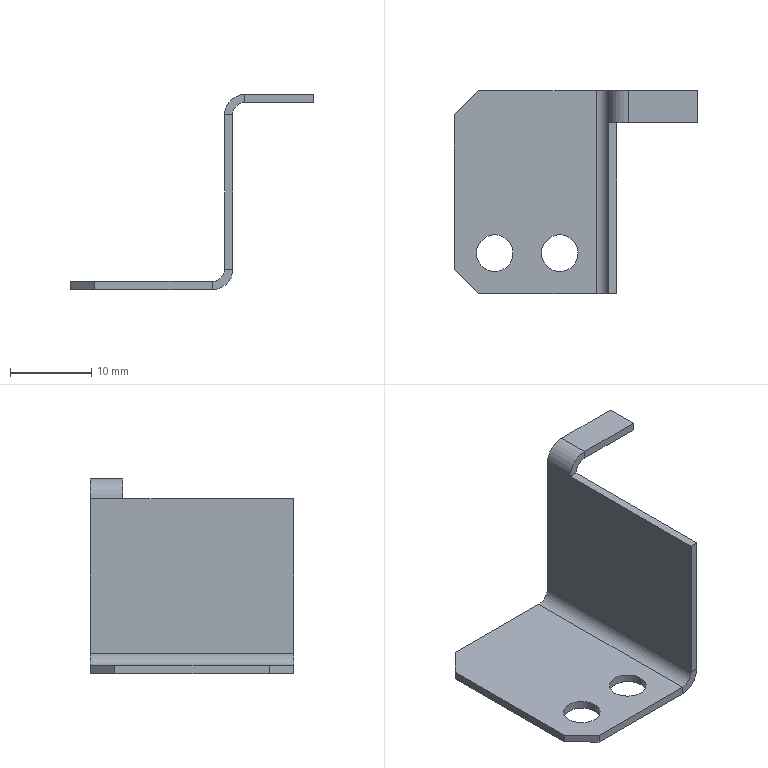Component | SolidWorks | F12529-S5108-2 | 1 solid | 29 faces | box 30 x 25 x 24 mm | volume 997 mm3 | plane 21 | cylinder 8 | commonest cylinder face diameters 4.5 x4 5 x2 3 x2
STEP:
#1=CARTESIAN_POINT('',(-1.467,7.795,1.201));
#2=VERTEX_POINT('',#1);
#3=CARTESIAN_POINT('',(-1.644,7.795,1.201));
#4=VERTEX_POINT('',#3);
#5=CARTESIAN_POINT('',(-1.555,7.795,1.201));
#6=DIRECTION('',(0.,0.,-1.));
#7=DIRECTION('',(-1.,0.,-0.));
#8=AXIS2_PLACEMENT_3D('',#5,#6,#7);
#9=CIRCLE('',#8,0.08858);
#10=EDGE_CURVE('',#2,#4,#9,.T.);
#11=ORIENTED_EDGE('',*,*,#10,.T.);
#12=CARTESIAN_POINT('',(-1.644,7.795,1.24));
#13=VERTEX_POINT('',#12);
#14=CARTESIAN_POINT('',(-1.644,7.795,0.8465));
#15=DIRECTION('',(-0.,0.,1.));
#16=VECTOR('',#15,39.37);
#17=LINE('',#14,#16);
#18=EDGE_CURVE('',#4,#13,#17,.T.);
#19=ORIENTED_EDGE('',*,*,#18,.T.);
#20=CARTESIAN_POINT('',(-1.467,7.795,1.24));
#21=VERTEX_POINT('',#20);
#22=CARTESIAN_POINT('',(-1.555,7.795,1.24));
#23=DIRECTION('',(-0.,0.,1.));
#24=DIRECTION('',(1.,0.,0.));
#25=AXIS2_PLACEMENT_3D('',#22,#23,#24);
#26=CIRCLE('',#25,0.08858);
#27=EDGE_CURVE('',#13,#21,#26,.T.);
#28=ORIENTED_EDGE('',*,*,#27,.T.);
#29=CARTESIAN_POINT('',(-1.467,7.795,0.8465));
#30=DIRECTION('',(-0.,0.,1.));
#31=VECTOR('',#30,39.37);
#32=LINE('',#29,#31);
#33=EDGE_CURVE('',#2,#21,#32,.T.);
#34=ORIENTED_EDGE('',*,*,#33,.F.);
#35=EDGE_LOOP('',(#11,#19,#28,#34));
#36=FACE_OUTER_BOUND('',#35,.T.);
#37=CARTESIAN_POINT('',(-1.555,7.795,0.8465));
#38=DIRECTION('',(-0.,0.,1.));
#39=DIRECTION('',(1.,0.,0.));
#40=AXIS2_PLACEMENT_3D('',#37,#38,#39);
#41=CYLINDRICAL_SURFACE('',#40,0.08858);
#42=ADVANCED_FACE('',(#36),#41,.F.);
#43=CARTESIAN_POINT('',(-1.781,7.795,1.201));
#44=VERTEX_POINT('',#43);
#45=CARTESIAN_POINT('',(-1.959,7.795,1.201));
#46=VERTEX_POINT('',#45);
#47=CARTESIAN_POINT('',(-1.87,7.795,1.201));
#48=DIRECTION('',(0.,0.,-1.));
#49=DIRECTION('',(-1.,0.,-0.));
#50=AXIS2_PLACEMENT_3D('',#47,#48,#49);
#51=CIRCLE('',#50,0.08858);
#52=EDGE_CURVE('',#44,#46,#51,.T.);
#53=ORIENTED_EDGE('',*,*,#52,.T.);
#54=CARTESIAN_POINT('',(-1.959,7.795,1.24));
#55=VERTEX_POINT('',#54);
#56=CARTESIAN_POINT('',(-1.959,7.795,0.8465));
#57=DIRECTION('',(-0.,0.,1.));
#58=VECTOR('',#57,39.37);
#59=LINE('',#56,#58);
#60=EDGE_CURVE('',#46,#55,#59,.T.);
#61=ORIENTED_EDGE('',*,*,#60,.T.);
#62=CARTESIAN_POINT('',(-1.781,7.795,1.24));
#63=VERTEX_POINT('',#62);
#64=CARTESIAN_POINT('',(-1.87,7.795,1.24));
#65=DIRECTION('',(-0.,0.,1.));
#66=DIRECTION('',(1.,0.,0.));
#67=AXIS2_PLACEMENT_3D('',#64,#65,#66);
#68=CIRCLE('',#67,0.08858);
#69=EDGE_CURVE('',#55,#63,#68,.T.);
#70=ORIENTED_EDGE('',*,*,#69,.T.);
#71=CARTESIAN_POINT('',(-1.781,7.795,0.8465));
#72=DIRECTION('',(-0.,0.,1.));
#73=VECTOR('',#72,39.37);
#74=LINE('',#71,#73);
#75=EDGE_CURVE('',#44,#63,#74,.T.);
#76=ORIENTED_EDGE('',*,*,#75,.F.);
#77=EDGE_LOOP('',(#53,#61,#70,#76));
#78=FACE_OUTER_BOUND('',#77,.T.);
#79=CARTESIAN_POINT('',(-1.87,7.795,0.8465));
#80=DIRECTION('',(-0.,0.,1.));
#81=DIRECTION('',(1.,0.,0.));
#82=AXIS2_PLACEMENT_3D('',#79,#80,#81);
#83=CYLINDRICAL_SURFACE('',#82,0.08858);
#84=ADVANCED_FACE('',(#78),#83,.F.);
#85=CARTESIAN_POINT('',(-1.28,8.583,1.299));
#86=VERTEX_POINT('',#85);
#87=CARTESIAN_POINT('',(-1.319,8.583,1.299));
#88=VERTEX_POINT('',#87);
#89=CARTESIAN_POINT('',(-1.28,8.583,1.299));
#90=DIRECTION('',(-1.,0.,-0.));
#91=VECTOR('',#90,39.37);
#92=LINE('',#89,#91);
#93=EDGE_CURVE('',#86,#88,#92,.T.);
#94=ORIENTED_EDGE('',*,*,#93,.F.);
#95=CARTESIAN_POINT('',(-1.378,8.583,1.201));
#96=VERTEX_POINT('',#95);
#97=CARTESIAN_POINT('',(-1.378,8.583,1.299));
#98=DIRECTION('',(0.,-1.,0.));
#99=DIRECTION('',(-1.,0.,0.));
#100=AXIS2_PLACEMENT_3D('',#97,#98,#99);
#101=CIRCLE('',#100,0.09843);
#102=EDGE_CURVE('',#96,#86,#101,.T.);
#103=ORIENTED_EDGE('',*,*,#102,.F.);
#104=CARTESIAN_POINT('',(-1.378,8.583,1.24));
#105=VERTEX_POINT('',#104);
#106=CARTESIAN_POINT('',(-1.378,8.583,1.24));
#107=DIRECTION('',(0.,0.,-1.));
#108=VECTOR('',#107,39.37);
#109=LINE('',#106,#108);
#110=EDGE_CURVE('',#105,#96,#109,.T.);
#111=ORIENTED_EDGE('',*,*,#110,.F.);
#112=CARTESIAN_POINT('',(-1.378,8.583,1.299));
#113=DIRECTION('',(0.,-1.,0.));
#114=DIRECTION('',(0.,0.,1.));
#115=AXIS2_PLACEMENT_3D('',#112,#113,#114);
#116=CIRCLE('',#115,0.05906);
#117=EDGE_CURVE('',#105,#88,#116,.T.);
#118=ORIENTED_EDGE('',*,*,#117,.T.);
#119=EDGE_LOOP('',(#94,#103,#111,#118));
#120=FACE_OUTER_BOUND('',#119,.T.);
#121=CARTESIAN_POINT('',(-1.28,8.583,1.299));
#122=DIRECTION('',(0.,1.,0.));
#123=DIRECTION('',(-1.,0.,-0.));
#124=AXIS2_PLACEMENT_3D('',#121,#122,#123);
#125=PLANE('',#124);
#126=ADVANCED_FACE('',(#120),#125,.T.);
#127=CARTESIAN_POINT('',(-1.28,8.583,2.047));
#128=VERTEX_POINT('',#127);
#129=CARTESIAN_POINT('',(-1.28,8.583,1.201));
#130=DIRECTION('',(-0.,0.,1.));
#131=VECTOR('',#130,39.37);
#132=LINE('',#129,#131);
#133=EDGE_CURVE('',#86,#128,#132,.T.);
#134=ORIENTED_EDGE('',*,*,#133,.F.);
#135=ORIENTED_EDGE('',*,*,#93,.T.);
#136=CARTESIAN_POINT('',(-1.319,8.583,2.047));
#137=VERTEX_POINT('',#136);
#138=CARTESIAN_POINT('',(-1.319,8.583,1.201));
#139=DIRECTION('',(-0.,0.,1.));
#140=VECTOR('',#139,39.37);
#141=LINE('',#138,#140);
#142=EDGE_CURVE('',#88,#137,#141,.T.);
#143=ORIENTED_EDGE('',*,*,#142,.T.);
#144=CARTESIAN_POINT('',(-1.319,8.583,2.047));
#145=DIRECTION('',(1.,0.,0.));
#146=VECTOR('',#145,39.37);
#147=LINE('',#144,#146);
#148=EDGE_CURVE('',#137,#128,#147,.T.);
#149=ORIENTED_EDGE('',*,*,#148,.T.);
#150=EDGE_LOOP('',(#134,#135,#143,#149));
#151=FACE_OUTER_BOUND('',#150,.T.);
#152=CARTESIAN_POINT('',(-1.378,8.583,1.24));
#153=DIRECTION('',(0.,1.,0.));
#154=DIRECTION('',(-1.,0.,-0.));
#155=AXIS2_PLACEMENT_3D('',#152,#153,#154);
#156=PLANE('',#155);
#157=ADVANCED_FACE('',(#151),#156,.T.);
#158=CARTESIAN_POINT('',(-1.378,7.598,1.201));
#159=VERTEX_POINT('',#158);
#160=CARTESIAN_POINT('',(-1.378,7.598,1.24));
#161=VERTEX_POINT('',#160);
#162=CARTESIAN_POINT('',(-1.378,7.598,1.201));
#163=DIRECTION('',(-0.,0.,1.));
#164=VECTOR('',#163,39.37);
#165=LINE('',#162,#164);
#166=EDGE_CURVE('',#159,#161,#165,.T.);
#167=ORIENTED_EDGE('',*,*,#166,.F.);
#168=CARTESIAN_POINT('',(-1.28,7.598,1.299));
#169=VERTEX_POINT('',#168);
#170=CARTESIAN_POINT('',(-1.378,7.598,1.299));
#171=DIRECTION('',(0.,-1.,0.));
#172=DIRECTION('',(-1.,0.,0.));
#173=AXIS2_PLACEMENT_3D('',#170,#171,#172);
#174=CIRCLE('',#173,0.09843);
#175=EDGE_CURVE('',#159,#169,#174,.T.);
#176=ORIENTED_EDGE('',*,*,#175,.T.);
#177=CARTESIAN_POINT('',(-1.319,7.598,1.299));
#178=VERTEX_POINT('',#177);
#179=CARTESIAN_POINT('',(-1.319,7.598,1.299));
#180=DIRECTION('',(1.,0.,0.));
#181=VECTOR('',#180,39.37);
#182=LINE('',#179,#181);
#183=EDGE_CURVE('',#178,#169,#182,.T.);
#184=ORIENTED_EDGE('',*,*,#183,.F.);
#185=CARTESIAN_POINT('',(-1.378,7.598,1.299));
#186=DIRECTION('',(0.,-1.,0.));
#187=DIRECTION('',(0.,0.,1.));
#188=AXIS2_PLACEMENT_3D('',#185,#186,#187);
#189=CIRCLE('',#188,0.05906);
#190=EDGE_CURVE('',#161,#178,#189,.T.);
#191=ORIENTED_EDGE('',*,*,#190,.F.);
#192=EDGE_LOOP('',(#167,#176,#184,#191));
#193=FACE_OUTER_BOUND('',#192,.T.);
#194=CARTESIAN_POINT('',(-1.378,7.598,1.201));
#195=DIRECTION('',(0.,-1.,0.));
#196=DIRECTION('',(1.,0.,0.));
#197=AXIS2_PLACEMENT_3D('',#194,#195,#196);
#198=PLANE('',#197);
#199=ADVANCED_FACE('',(#193),#198,.T.);
#200=CARTESIAN_POINT('',(-1.949,7.598,1.24));
#201=VERTEX_POINT('',#200);
#202=CARTESIAN_POINT('',(-2.067,7.598,1.24));
#203=DIRECTION('',(1.,0.,0.));
#204=VECTOR('',#203,39.37);
#205=LINE('',#202,#204);
#206=EDGE_CURVE('',#201,#161,#205,.T.);
#207=ORIENTED_EDGE('',*,*,#206,.F.);
#208=CARTESIAN_POINT('',(-1.949,7.598,1.201));
#209=VERTEX_POINT('',#208);
#210=CARTESIAN_POINT('',(-1.949,7.598,1.299));
#211=DIRECTION('',(0.,0.,-1.));
#212=VECTOR('',#211,39.37);
#213=LINE('',#210,#212);
#214=EDGE_CURVE('',#201,#209,#213,.T.);
#215=ORIENTED_EDGE('',*,*,#214,.T.);
#216=CARTESIAN_POINT('',(-2.067,7.598,1.201));
#217=DIRECTION('',(1.,0.,0.));
#218=VECTOR('',#217,39.37);
#219=LINE('',#216,#218);
#220=EDGE_CURVE('',#209,#159,#219,.T.);
#221=ORIENTED_EDGE('',*,*,#220,.T.);
#222=ORIENTED_EDGE('',*,*,#166,.T.);
#223=EDGE_LOOP('',(#207,#215,#221,#222));
#224=FACE_OUTER_BOUND('',#223,.T.);
#225=CARTESIAN_POINT('',(-1.319,7.598,1.299));
#226=DIRECTION('',(0.,-1.,0.));
#227=DIRECTION('',(1.,0.,0.));
#228=AXIS2_PLACEMENT_3D('',#225,#226,#227);
#229=PLANE('',#228);
#230=ADVANCED_FACE('',(#224),#229,.T.);
#231=CARTESIAN_POINT('',(-1.28,7.598,2.047));
#232=VERTEX_POINT('',#231);
#233=CARTESIAN_POINT('',(-1.28,7.598,1.201));
#234=DIRECTION('',(-0.,0.,1.));
#235=VECTOR('',#234,39.37);
#236=LINE('',#233,#235);
#237=EDGE_CURVE('',#169,#232,#236,.T.);
#238=ORIENTED_EDGE('',*,*,#237,.T.);
#239=CARTESIAN_POINT('',(-1.319,7.598,2.047));
#240=VERTEX_POINT('',#239);
#241=CARTESIAN_POINT('',(-1.28,7.598,2.047));
#242=DIRECTION('',(-1.,0.,-0.));
#243=VECTOR('',#242,39.37);
#244=LINE('',#241,#243);
#245=EDGE_CURVE('',#232,#240,#244,.T.);
#246=ORIENTED_EDGE('',*,*,#245,.T.);
#247=CARTESIAN_POINT('',(-1.319,7.598,1.201));
#248=DIRECTION('',(-0.,0.,1.));
#249=VECTOR('',#248,39.37);
#250=LINE('',#247,#249);
#251=EDGE_CURVE('',#178,#240,#250,.T.);
#252=ORIENTED_EDGE('',*,*,#251,.F.);
#253=ORIENTED_EDGE('',*,*,#183,.T.);
#254=EDGE_LOOP('',(#238,#246,#252,#253));
#255=FACE_OUTER_BOUND('',#254,.T.);
#256=CARTESIAN_POINT('',(-1.22,7.598,2.146));
#257=DIRECTION('',(0.,-1.,0.));
#258=DIRECTION('',(1.,0.,0.));
#259=AXIS2_PLACEMENT_3D('',#256,#257,#258);
#260=PLANE('',#259);
#261=ADVANCED_FACE('',(#255),#260,.T.);
#262=ORIENTED_EDGE('',*,*,#237,.F.);
#263=CARTESIAN_POINT('',(-1.28,8.583,1.299));
#264=DIRECTION('',(0.,-1.,0.));
#265=VECTOR('',#264,39.37);
#266=LINE('',#263,#265);
#267=EDGE_CURVE('',#86,#169,#266,.T.);
#268=ORIENTED_EDGE('',*,*,#267,.F.);
#269=ORIENTED_EDGE('',*,*,#133,.T.);
#270=CARTESIAN_POINT('',(-1.28,8.425,2.047));
#271=VERTEX_POINT('',#270);
#272=CARTESIAN_POINT('',(-1.28,8.583,2.047));
#273=DIRECTION('',(0.,-1.,0.));
#274=VECTOR('',#273,39.37);
#275=LINE('',#272,#274);
#276=EDGE_CURVE('',#128,#271,#275,.T.);
#277=ORIENTED_EDGE('',*,*,#276,.T.);
#278=CARTESIAN_POINT('',(-1.28,7.598,2.047));
#279=DIRECTION('',(0.,-1.,0.));
#280=VECTOR('',#279,39.37);
#281=LINE('',#278,#280);
#282=EDGE_CURVE('',#271,#232,#281,.T.);
#283=ORIENTED_EDGE('',*,*,#282,.T.);
#284=EDGE_LOOP('',(#262,#268,#269,#277,#283));
#285=FACE_OUTER_BOUND('',#284,.T.);
#286=CARTESIAN_POINT('',(-1.28,8.583,1.201));
#287=DIRECTION('',(1.,0.,0.));
#288=DIRECTION('',(0.,0.,-1.));
#289=AXIS2_PLACEMENT_3D('',#286,#287,#288);
#290=PLANE('',#289);
#291=ADVANCED_FACE('',(#285),#290,.T.);
#292=ORIENTED_EDGE('',*,*,#175,.F.);
#293=CARTESIAN_POINT('',(-1.378,8.583,1.201));
#294=DIRECTION('',(0.,-1.,0.));
#295=VECTOR('',#294,39.37);
#296=LINE('',#293,#295);
#297=EDGE_CURVE('',#96,#159,#296,.T.);
#298=ORIENTED_EDGE('',*,*,#297,.F.);
#299=ORIENTED_EDGE('',*,*,#102,.T.);
#300=ORIENTED_EDGE('',*,*,#267,.T.);
#301=EDGE_LOOP('',(#292,#298,#299,#300));
#302=FACE_OUTER_BOUND('',#301,.T.);
#303=CARTESIAN_POINT('',(-1.378,8.583,1.299));
#304=DIRECTION('',(0.,-1.,0.));
#305=DIRECTION('',(1.,0.,0.));
#306=AXIS2_PLACEMENT_3D('',#303,#304,#305);
#307=CYLINDRICAL_SURFACE('',#306,0.09843);
#308=ADVANCED_FACE('',(#302),#307,.T.);
#309=ORIENTED_EDGE('',*,*,#10,.F.);
#310=CARTESIAN_POINT('',(-1.555,7.795,1.201));
#311=DIRECTION('',(0.,0.,-1.));
#312=DIRECTION('',(-1.,0.,-0.));
#313=AXIS2_PLACEMENT_3D('',#310,#311,#312);
#314=CIRCLE('',#313,0.08858);
#315=EDGE_CURVE('',#4,#2,#314,.T.);
#316=ORIENTED_EDGE('',*,*,#315,.F.);
#317=EDGE_LOOP('',(#309,#316));
#318=FACE_BOUND('',#317,.T.);
#319=ORIENTED_EDGE('',*,*,#52,.F.);
#320=CARTESIAN_POINT('',(-1.87,7.795,1.201));
#321=DIRECTION('',(0.,0.,-1.));
#322=DIRECTION('',(-1.,0.,-0.));
#323=AXIS2_PLACEMENT_3D('',#320,#321,#322);
#324=CIRCLE('',#323,0.08858);
#325=EDGE_CURVE('',#46,#44,#324,.T.);
#326=ORIENTED_EDGE('',*,*,#325,.F.);
#327=EDGE_LOOP('',(#319,#326));
#328=FACE_BOUND('',#327,.T.);
#329=ORIENTED_EDGE('',*,*,#220,.F.);
#330=CARTESIAN_POINT('',(-2.067,7.717,1.201));
#331=VERTEX_POINT('',#330);
#332=CARTESIAN_POINT('',(-2.5,8.15,1.201));
#333=DIRECTION('',(-0.7071,0.7071,-0.));
#334=VECTOR('',#333,39.37);
#335=LINE('',#332,#334);
#336=EDGE_CURVE('',#209,#331,#335,.T.);
#337=ORIENTED_EDGE('',*,*,#336,.T.);
#338=CARTESIAN_POINT('',(-2.067,8.465,1.201));
#339=VERTEX_POINT('',#338);
#340=CARTESIAN_POINT('',(-2.067,8.583,1.201));
#341=DIRECTION('',(0.,-1.,0.));
#342=VECTOR('',#341,39.37);
#343=LINE('',#340,#342);
#344=EDGE_CURVE('',#339,#331,#343,.T.);
#345=ORIENTED_EDGE('',*,*,#344,.F.);
#346=CARTESIAN_POINT('',(-1.949,8.583,1.201));
#347=VERTEX_POINT('',#346);
#348=CARTESIAN_POINT('',(-2.008,8.524,1.201));
#349=DIRECTION('',(0.7071,0.7071,0.));
#350=VECTOR('',#349,39.37);
#351=LINE('',#348,#350);
#352=EDGE_CURVE('',#339,#347,#351,.T.);
#353=ORIENTED_EDGE('',*,*,#352,.T.);
#354=CARTESIAN_POINT('',(-2.067,8.583,1.201));
#355=DIRECTION('',(1.,0.,0.));
#356=VECTOR('',#355,39.37);
#357=LINE('',#354,#356);
#358=EDGE_CURVE('',#347,#96,#357,.T.);
#359=ORIENTED_EDGE('',*,*,#358,.T.);
#360=ORIENTED_EDGE('',*,*,#297,.T.);
#361=EDGE_LOOP('',(#329,#337,#345,#353,#359,#360));
#362=FACE_OUTER_BOUND('',#361,.T.);
#363=CARTESIAN_POINT('',(-2.067,8.583,1.201));
#364=DIRECTION('',(0.,0.,-1.));
#365=DIRECTION('',(-1.,0.,-0.));
#366=AXIS2_PLACEMENT_3D('',#363,#364,#365);
#367=PLANE('',#366);
#368=ADVANCED_FACE('',(#318,#328,#362),#367,.T.);
#369=ORIENTED_EDGE('',*,*,#344,.T.);
#370=CARTESIAN_POINT('',(-2.067,7.717,1.24));
#371=VERTEX_POINT('',#370);
#372=CARTESIAN_POINT('',(-2.067,7.717,1.24));
#373=DIRECTION('',(-0.,0.,1.));
#374=VECTOR('',#373,39.37);
#375=LINE('',#372,#374);
#376=EDGE_CURVE('',#331,#371,#375,.T.);
#377=ORIENTED_EDGE('',*,*,#376,.T.);
#378=CARTESIAN_POINT('',(-2.067,8.465,1.24));
#379=VERTEX_POINT('',#378);
#380=CARTESIAN_POINT('',(-2.067,8.583,1.24));
#381=DIRECTION('',(0.,-1.,0.));
#382=VECTOR('',#381,39.37);
#383=LINE('',#380,#382);
#384=EDGE_CURVE('',#379,#371,#383,.T.);
#385=ORIENTED_EDGE('',*,*,#384,.F.);
#386=CARTESIAN_POINT('',(-2.067,8.465,1.201));
#387=DIRECTION('',(0.,0.,-1.));
#388=VECTOR('',#387,39.37);
#389=LINE('',#386,#388);
#390=EDGE_CURVE('',#379,#339,#389,.T.);
#391=ORIENTED_EDGE('',*,*,#390,.T.);
#392=EDGE_LOOP('',(#369,#377,#385,#391));
#393=FACE_OUTER_BOUND('',#392,.T.);
#394=CARTESIAN_POINT('',(-2.067,8.583,1.24));
#395=DIRECTION('',(-1.,0.,-0.));
#396=DIRECTION('',(-0.,0.,1.));
#397=AXIS2_PLACEMENT_3D('',#394,#395,#396);
#398=PLANE('',#397);
#399=ADVANCED_FACE('',(#393),#398,.T.);
#400=CARTESIAN_POINT('',(-1.555,7.795,1.24));
#401=DIRECTION('',(-0.,0.,1.));
#402=DIRECTION('',(1.,0.,0.));
#403=AXIS2_PLACEMENT_3D('',#400,#401,#402);
#404=CIRCLE('',#403,0.08858);
#405=EDGE_CURVE('',#21,#13,#404,.T.);
#406=ORIENTED_EDGE('',*,*,#405,.F.);
#407=ORIENTED_EDGE('',*,*,#27,.F.);
#408=EDGE_LOOP('',(#406,#407));
#409=FACE_BOUND('',#408,.T.);
#410=CARTESIAN_POINT('',(-1.87,7.795,1.24));
#411=DIRECTION('',(-0.,0.,1.));
#412=DIRECTION('',(1.,0.,0.));
#413=AXIS2_PLACEMENT_3D('',#410,#411,#412);
#414=CIRCLE('',#413,0.08858);
#415=EDGE_CURVE('',#63,#55,#414,.T.);
#416=ORIENTED_EDGE('',*,*,#415,.F.);
#417=ORIENTED_EDGE('',*,*,#69,.F.);
#418=EDGE_LOOP('',(#416,#417));
#419=FACE_BOUND('',#418,.T.);
#420=ORIENTED_EDGE('',*,*,#384,.T.);
#421=CARTESIAN_POINT('',(-1.949,7.598,1.24));
#422=DIRECTION('',(0.7071,-0.7071,0.));
#423=VECTOR('',#422,39.37);
#424=LINE('',#421,#423);
#425=EDGE_CURVE('',#371,#201,#424,.T.);
#426=ORIENTED_EDGE('',*,*,#425,.T.);
#427=ORIENTED_EDGE('',*,*,#206,.T.);
#428=CARTESIAN_POINT('',(-1.378,8.583,1.24));
#429=DIRECTION('',(0.,-1.,0.));
#430=VECTOR('',#429,39.37);
#431=LINE('',#428,#430);
#432=EDGE_CURVE('',#105,#161,#431,.T.);
#433=ORIENTED_EDGE('',*,*,#432,.F.);
#434=CARTESIAN_POINT('',(-1.949,8.583,1.24));
#435=VERTEX_POINT('',#434);
#436=CARTESIAN_POINT('',(-2.067,8.583,1.24));
#437=DIRECTION('',(1.,0.,0.));
#438=VECTOR('',#437,39.37);
#439=LINE('',#436,#438);
#440=EDGE_CURVE('',#435,#105,#439,.T.);
#441=ORIENTED_EDGE('',*,*,#440,.F.);
#442=CARTESIAN_POINT('',(-2.067,8.465,1.24));
#443=DIRECTION('',(-0.7071,-0.7071,-0.));
#444=VECTOR('',#443,39.37);
#445=LINE('',#442,#444);
#446=EDGE_CURVE('',#435,#379,#445,.T.);
#447=ORIENTED_EDGE('',*,*,#446,.T.);
#448=EDGE_LOOP('',(#420,#426,#427,#433,#441,#447));
#449=FACE_OUTER_BOUND('',#448,.T.);
#450=CARTESIAN_POINT('',(-2.067,8.583,1.24));
#451=DIRECTION('',(0.,0.,-1.));
#452=DIRECTION('',(-1.,0.,-0.));
#453=AXIS2_PLACEMENT_3D('',#450,#451,#452);
#454=PLANE('',#453);
#455=ADVANCED_FACE('',(#409,#419,#449),#454,.F.);
#456=ORIENTED_EDGE('',*,*,#190,.T.);
#457=CARTESIAN_POINT('',(-1.319,8.583,1.299));
#458=DIRECTION('',(0.,-1.,0.));
#459=VECTOR('',#458,39.37);
#460=LINE('',#457,#459);
#461=EDGE_CURVE('',#88,#178,#460,.T.);
#462=ORIENTED_EDGE('',*,*,#461,.F.);
#463=ORIENTED_EDGE('',*,*,#117,.F.);
#464=ORIENTED_EDGE('',*,*,#432,.T.);
#465=EDGE_LOOP('',(#456,#462,#463,#464));
#466=FACE_OUTER_BOUND('',#465,.T.);
#467=CARTESIAN_POINT('',(-1.378,8.583,1.299));
#468=DIRECTION('',(0.,-1.,0.));
#469=DIRECTION('',(1.,0.,0.));
#470=AXIS2_PLACEMENT_3D('',#467,#468,#469);
#471=CYLINDRICAL_SURFACE('',#470,0.05906);
#472=ADVANCED_FACE('',(#466),#471,.F.);
#473=ORIENTED_EDGE('',*,*,#251,.T.);
#474=CARTESIAN_POINT('',(-1.319,8.425,2.047));
#475=VERTEX_POINT('',#474);
#476=CARTESIAN_POINT('',(-1.319,7.598,2.047));
#477=DIRECTION('',(0.,-1.,0.));
#478=VECTOR('',#477,39.37);
#479=LINE('',#476,#478);
#480=EDGE_CURVE('',#475,#240,#479,.T.);
#481=ORIENTED_EDGE('',*,*,#480,.F.);
#482=CARTESIAN_POINT('',(-1.319,8.583,2.047));
#483=DIRECTION('',(0.,-1.,0.));
#484=VECTOR('',#483,39.37);
#485=LINE('',#482,#484);
#486=EDGE_CURVE('',#137,#475,#485,.T.);
#487=ORIENTED_EDGE('',*,*,#486,.F.);
#488=ORIENTED_EDGE('',*,*,#142,.F.);
#489=ORIENTED_EDGE('',*,*,#461,.T.);
#490=EDGE_LOOP('',(#473,#481,#487,#488,#489));
#491=FACE_OUTER_BOUND('',#490,.T.);
#492=CARTESIAN_POINT('',(-1.319,8.583,1.201));
#493=DIRECTION('',(1.,0.,0.));
#494=DIRECTION('',(0.,0.,-1.));
#495=AXIS2_PLACEMENT_3D('',#492,#493,#494);
#496=PLANE('',#495);
#497=ADVANCED_FACE('',(#491),#496,.F.);
#498=ORIENTED_EDGE('',*,*,#358,.F.);
#499=CARTESIAN_POINT('',(-1.949,8.583,1.24));
#500=DIRECTION('',(-0.,0.,1.));
#501=VECTOR('',#500,39.37);
#502=LINE('',#499,#501);
#503=EDGE_CURVE('',#347,#435,#502,.T.);
#504=ORIENTED_EDGE('',*,*,#503,.T.);
#505=ORIENTED_EDGE('',*,*,#440,.T.);
#506=ORIENTED_EDGE('',*,*,#110,.T.);
#507=EDGE_LOOP('',(#498,#504,#505,#506));
#508=FACE_OUTER_BOUND('',#507,.T.);
#509=CARTESIAN_POINT('',(-1.22,8.583,2.047));
#510=DIRECTION('',(0.,-1.,0.));
#511=DIRECTION('',(0.,0.,-1.));
#512=AXIS2_PLACEMENT_3D('',#509,#510,#511);
#513=PLANE('',#512);
#514=ADVANCED_FACE('',(#508),#513,.F.);
#515=ORIENTED_EDGE('',*,*,#425,.F.);
#516=ORIENTED_EDGE('',*,*,#376,.F.);
#517=ORIENTED_EDGE('',*,*,#336,.F.);
#518=ORIENTED_EDGE('',*,*,#214,.F.);
#519=EDGE_LOOP('',(#515,#516,#517,#518));
#520=FACE_OUTER_BOUND('',#519,.T.);
#521=CARTESIAN_POINT('',(-1.949,7.598,1.299));
#522=DIRECTION('',(0.7071,0.7071,0.));
#523=DIRECTION('',(-0.7071,0.7071,-0.));
#524=AXIS2_PLACEMENT_3D('',#521,#522,#523);
#525=PLANE('',#524);
#526=ADVANCED_FACE('',(#520),#525,.F.);
#527=ORIENTED_EDGE('',*,*,#446,.F.);
#528=ORIENTED_EDGE('',*,*,#503,.F.);
#529=ORIENTED_EDGE('',*,*,#352,.F.);
#530=ORIENTED_EDGE('',*,*,#390,.F.);
#531=EDGE_LOOP('',(#527,#528,#529,#530));
#532=FACE_OUTER_BOUND('',#531,.T.);
#533=CARTESIAN_POINT('',(-2.067,8.465,1.24));
#534=DIRECTION('',(-0.7071,0.7071,-0.));
#535=DIRECTION('',(-0.7071,-0.7071,-0.));
#536=AXIS2_PLACEMENT_3D('',#533,#534,#535);
#537=PLANE('',#536);
#538=ADVANCED_FACE('',(#532),#537,.T.);
#539=ORIENTED_EDGE('',*,*,#480,.T.);
#540=ORIENTED_EDGE('',*,*,#245,.F.);
#541=ORIENTED_EDGE('',*,*,#282,.F.);
#542=CARTESIAN_POINT('',(-1.28,8.425,2.047));
#543=DIRECTION('',(-1.,0.,-0.));
#544=VECTOR('',#543,39.37);
#545=LINE('',#542,#544);
#546=EDGE_CURVE('',#271,#475,#545,.T.);
#547=ORIENTED_EDGE('',*,*,#546,.T.);
#548=EDGE_LOOP('',(#539,#540,#541,#547));
#549=FACE_OUTER_BOUND('',#548,.T.);
#550=CARTESIAN_POINT('',(-1.28,7.598,2.047));
#551=DIRECTION('',(0.,0.,-1.));
#552=DIRECTION('',(-1.,0.,-0.));
#553=AXIS2_PLACEMENT_3D('',#550,#551,#552);
#554=PLANE('',#553);
#555=ADVANCED_FACE('',(#549),#554,.F.);
#556=CARTESIAN_POINT('',(-1.22,8.425,2.106));
#557=VERTEX_POINT('',#556);
#558=CARTESIAN_POINT('',(-1.22,8.425,2.146));
#559=VERTEX_POINT('',#558);
#560=CARTESIAN_POINT('',(-1.22,8.425,2.106));
#561=DIRECTION('',(-0.,0.,1.));
#562=VECTOR('',#561,39.37);
#563=LINE('',#560,#562);
#564=EDGE_CURVE('',#557,#559,#563,.T.);
#565=ORIENTED_EDGE('',*,*,#564,.T.);
#566=CARTESIAN_POINT('',(-1.22,8.425,2.047));
#567=DIRECTION('',(0.,-1.,0.));
#568=DIRECTION('',(1.,0.,0.));
#569=AXIS2_PLACEMENT_3D('',#566,#567,#568);
#570=CIRCLE('',#569,0.09843);
#571=EDGE_CURVE('',#559,#475,#570,.T.);
#572=ORIENTED_EDGE('',*,*,#571,.T.);
#573=ORIENTED_EDGE('',*,*,#546,.F.);
#574=CARTESIAN_POINT('',(-1.22,8.425,2.047));
#575=DIRECTION('',(0.,-1.,0.));
#576=DIRECTION('',(1.,0.,0.));
#577=AXIS2_PLACEMENT_3D('',#574,#575,#576);
#578=CIRCLE('',#577,0.05906);
#579=EDGE_CURVE('',#557,#271,#578,.T.);
#580=ORIENTED_EDGE('',*,*,#579,.F.);
#581=EDGE_LOOP('',(#565,#572,#573,#580));
#582=FACE_OUTER_BOUND('',#581,.T.);
#583=CARTESIAN_POINT('',(-1.22,8.425,2.047));
#584=DIRECTION('',(0.,1.,0.));
#585=DIRECTION('',(-1.,0.,-0.));
#586=AXIS2_PLACEMENT_3D('',#583,#584,#585);
#587=PLANE('',#586);
#588=ADVANCED_FACE('',(#582),#587,.F.);
#589=ORIENTED_EDGE('',*,*,#148,.F.);
#590=CARTESIAN_POINT('',(-1.22,8.583,2.146));
#591=VERTEX_POINT('',#590);
#592=CARTESIAN_POINT('',(-1.22,8.583,2.047));
#593=DIRECTION('',(0.,1.,0.));
#594=DIRECTION('',(1.,0.,0.));
#595=AXIS2_PLACEMENT_3D('',#592,#593,#594);
#596=CIRCLE('',#595,0.09843);
#597=EDGE_CURVE('',#137,#591,#596,.T.);
#598=ORIENTED_EDGE('',*,*,#597,.T.);
#599=CARTESIAN_POINT('',(-1.22,8.583,2.106));
#600=VERTEX_POINT('',#599);
#601=CARTESIAN_POINT('',(-1.22,8.583,2.106));
#602=DIRECTION('',(-0.,0.,1.));
#603=VECTOR('',#602,39.37);
#604=LINE('',#601,#603);
#605=EDGE_CURVE('',#600,#591,#604,.T.);
#606=ORIENTED_EDGE('',*,*,#605,.F.);
#607=CARTESIAN_POINT('',(-1.22,8.583,2.047));
#608=DIRECTION('',(0.,1.,0.));
#609=DIRECTION('',(-1.,0.,0.));
#610=AXIS2_PLACEMENT_3D('',#607,#608,#609);
#611=CIRCLE('',#610,0.05906);
#612=EDGE_CURVE('',#128,#600,#611,.T.);
#613=ORIENTED_EDGE('',*,*,#612,.F.);
#614=EDGE_LOOP('',(#589,#598,#606,#613));
#615=FACE_OUTER_BOUND('',#614,.T.);
#616=CARTESIAN_POINT('',(-1.22,8.583,2.047));
#617=DIRECTION('',(0.,-1.,0.));
#618=DIRECTION('',(1.,0.,0.));
#619=AXIS2_PLACEMENT_3D('',#616,#617,#618);
#620=PLANE('',#619);
#621=ADVANCED_FACE('',(#615),#620,.F.);
#622=ORIENTED_EDGE('',*,*,#612,.T.);
#623=CARTESIAN_POINT('',(-1.22,8.583,2.106));
#624=DIRECTION('',(0.,-1.,0.));
#625=VECTOR('',#624,39.37);
#626=LINE('',#623,#625);
#627=EDGE_CURVE('',#600,#557,#626,.T.);
#628=ORIENTED_EDGE('',*,*,#627,.T.);
#629=ORIENTED_EDGE('',*,*,#579,.T.);
#630=ORIENTED_EDGE('',*,*,#276,.F.);
#631=EDGE_LOOP('',(#622,#628,#629,#630));
#632=FACE_OUTER_BOUND('',#631,.T.);
#633=CARTESIAN_POINT('',(-1.22,8.708,2.047));
#634=DIRECTION('',(0.,-1.,0.));
#635=DIRECTION('',(1.,0.,0.));
#636=AXIS2_PLACEMENT_3D('',#633,#634,#635);
#637=CYLINDRICAL_SURFACE('',#636,0.05906);
#638=ADVANCED_FACE('',(#632),#637,.F.);
#639=ORIENTED_EDGE('',*,*,#597,.F.);
#640=ORIENTED_EDGE('',*,*,#486,.T.);
#641=ORIENTED_EDGE('',*,*,#571,.F.);
#642=CARTESIAN_POINT('',(-1.22,8.583,2.146));
#643=DIRECTION('',(0.,-1.,0.));
#644=VECTOR('',#643,39.37);
#645=LINE('',#642,#644);
#646=EDGE_CURVE('',#591,#559,#645,.T.);
#647=ORIENTED_EDGE('',*,*,#646,.F.);
#648=EDGE_LOOP('',(#639,#640,#641,#647));
#649=FACE_OUTER_BOUND('',#648,.T.);
#650=CARTESIAN_POINT('',(-1.22,8.708,2.047));
#651=DIRECTION('',(0.,-1.,0.));
#652=DIRECTION('',(1.,0.,0.));
#653=AXIS2_PLACEMENT_3D('',#650,#651,#652);
#654=CYLINDRICAL_SURFACE('',#653,0.09843);
#655=ADVANCED_FACE('',(#649),#654,.T.);
#656=CARTESIAN_POINT('',(-0.8858,8.425,2.106));
#657=VERTEX_POINT('',#656);
#658=CARTESIAN_POINT('',(-0.8858,8.425,2.146));
#659=VERTEX_POINT('',#658);
#660=CARTESIAN_POINT('',(-0.8858,8.425,2.106));
#661=DIRECTION('',(-0.,0.,1.));
#662=VECTOR('',#661,39.37);
#663=LINE('',#660,#662);
#664=EDGE_CURVE('',#657,#659,#663,.T.);
#665=ORIENTED_EDGE('',*,*,#664,.F.);
#666=CARTESIAN_POINT('',(-0.8858,8.583,2.106));
#667=VERTEX_POINT('',#666);
#668=CARTESIAN_POINT('',(-0.8858,8.583,2.106));
#669=DIRECTION('',(0.,-1.,0.));
#670=VECTOR('',#669,39.37);
#671=LINE('',#668,#670);
#672=EDGE_CURVE('',#667,#657,#671,.T.);
#673=ORIENTED_EDGE('',*,*,#672,.F.);
#674=CARTESIAN_POINT('',(-0.8858,8.583,2.146));
#675=VERTEX_POINT('',#674);
#676=CARTESIAN_POINT('',(-0.8858,8.583,2.106));
#677=DIRECTION('',(-0.,0.,1.));
#678=VECTOR('',#677,39.37);
#679=LINE('',#676,#678);
#680=EDGE_CURVE('',#667,#675,#679,.T.);
#681=ORIENTED_EDGE('',*,*,#680,.T.);
#682=CARTESIAN_POINT('',(-0.8858,8.583,2.146));
#683=DIRECTION('',(0.,-1.,0.));
#684=VECTOR('',#683,39.37);
#685=LINE('',#682,#684);
#686=EDGE_CURVE('',#675,#659,#685,.T.);
#687=ORIENTED_EDGE('',*,*,#686,.T.);
#688=EDGE_LOOP('',(#665,#673,#681,#687));
#689=FACE_OUTER_BOUND('',#688,.T.);
#690=CARTESIAN_POINT('',(-0.8858,8.583,2.106));
#691=DIRECTION('',(1.,0.,0.));
#692=DIRECTION('',(0.,0.,-1.));
#693=AXIS2_PLACEMENT_3D('',#690,#691,#692);
#694=PLANE('',#693);
#695=ADVANCED_FACE('',(#689),#694,.T.);
#696=CARTESIAN_POINT('',(-0.8858,8.425,2.106));
#697=DIRECTION('',(-1.,-0.,-0.));
#698=VECTOR('',#697,39.37);
#699=LINE('',#696,#698);
#700=EDGE_CURVE('',#657,#557,#699,.T.);
#701=ORIENTED_EDGE('',*,*,#700,.T.);
#702=ORIENTED_EDGE('',*,*,#627,.F.);
#703=CARTESIAN_POINT('',(-1.28,8.583,2.106));
#704=DIRECTION('',(1.,0.,0.));
#705=VECTOR('',#704,39.37);
#706=LINE('',#703,#705);
#707=EDGE_CURVE('',#600,#667,#706,.T.);
#708=ORIENTED_EDGE('',*,*,#707,.T.);
#709=ORIENTED_EDGE('',*,*,#672,.T.);
#710=EDGE_LOOP('',(#701,#702,#708,#709));
#711=FACE_OUTER_BOUND('',#710,.T.);
#712=CARTESIAN_POINT('',(-1.28,8.583,2.106));
#713=DIRECTION('',(0.,0.,-1.));
#714=DIRECTION('',(-1.,0.,-0.));
#715=AXIS2_PLACEMENT_3D('',#712,#713,#714);
#716=PLANE('',#715);
#717=ADVANCED_FACE('',(#711),#716,.T.);
#718=ORIENTED_EDGE('',*,*,#707,.F.);
#719=ORIENTED_EDGE('',*,*,#605,.T.);
#720=CARTESIAN_POINT('',(-1.28,8.583,2.146));
#721=DIRECTION('',(1.,0.,0.));
#722=VECTOR('',#721,39.37);
#723=LINE('',#720,#722);
#724=EDGE_CURVE('',#591,#675,#723,.T.);
#725=ORIENTED_EDGE('',*,*,#724,.T.);
#726=ORIENTED_EDGE('',*,*,#680,.F.);
#727=EDGE_LOOP('',(#718,#719,#725,#726));
#728=FACE_OUTER_BOUND('',#727,.T.);
#729=CARTESIAN_POINT('',(-1.319,8.583,2.047));
#730=DIRECTION('',(0.,1.,0.));
#731=DIRECTION('',(-1.,0.,-0.));
#732=AXIS2_PLACEMENT_3D('',#729,#730,#731);
#733=PLANE('',#732);
#734=ADVANCED_FACE('',(#728),#733,.T.);
#735=ORIENTED_EDGE('',*,*,#646,.T.);
#736=CARTESIAN_POINT('',(-0.8858,8.425,2.146));
#737=DIRECTION('',(-1.,-0.,-0.));
#738=VECTOR('',#737,39.37);
#739=LINE('',#736,#738);
#740=EDGE_CURVE('',#659,#559,#739,.T.);
#741=ORIENTED_EDGE('',*,*,#740,.F.);
#742=ORIENTED_EDGE('',*,*,#686,.F.);
#743=ORIENTED_EDGE('',*,*,#724,.F.);
#744=EDGE_LOOP('',(#735,#741,#742,#743));
#745=FACE_OUTER_BOUND('',#744,.T.);
#746=CARTESIAN_POINT('',(-1.28,8.583,2.146));
#747=DIRECTION('',(0.,0.,-1.));
#748=DIRECTION('',(-1.,0.,-0.));
#749=AXIS2_PLACEMENT_3D('',#746,#747,#748);
#750=PLANE('',#749);
#751=ADVANCED_FACE('',(#745),#750,.F.);
#752=ORIENTED_EDGE('',*,*,#564,.F.);
#753=ORIENTED_EDGE('',*,*,#700,.F.);
#754=ORIENTED_EDGE('',*,*,#664,.T.);
#755=ORIENTED_EDGE('',*,*,#740,.T.);
#756=EDGE_LOOP('',(#752,#753,#754,#755));
#757=FACE_OUTER_BOUND('',#756,.T.);
#758=CARTESIAN_POINT('',(-0.8858,8.425,2.106));
#759=DIRECTION('',(-0.,1.,-0.));
#760=DIRECTION('',(-1.,-0.,-0.));
#761=AXIS2_PLACEMENT_3D('',#758,#759,#760);
#762=PLANE('',#761);
#763=ADVANCED_FACE('',(#757),#762,.F.);
#764=ORIENTED_EDGE('',*,*,#60,.F.);
#765=ORIENTED_EDGE('',*,*,#325,.T.);
#766=ORIENTED_EDGE('',*,*,#75,.T.);
#767=ORIENTED_EDGE('',*,*,#415,.T.);
#768=EDGE_LOOP('',(#764,#765,#766,#767));
#769=FACE_OUTER_BOUND('',#768,.T.);
#770=CARTESIAN_POINT('',(-1.87,7.795,0.8465));
#771=DIRECTION('',(-0.,0.,1.));
#772=DIRECTION('',(1.,0.,0.));
#773=AXIS2_PLACEMENT_3D('',#770,#771,#772);
#774=CYLINDRICAL_SURFACE('',#773,0.08858);
#775=ADVANCED_FACE('',(#769),#774,.F.);
#776=ORIENTED_EDGE('',*,*,#18,.F.);
#777=ORIENTED_EDGE('',*,*,#315,.T.);
#778=ORIENTED_EDGE('',*,*,#33,.T.);
#779=ORIENTED_EDGE('',*,*,#405,.T.);
#780=EDGE_LOOP('',(#776,#777,#778,#779));
#781=FACE_OUTER_BOUND('',#780,.T.);
#782=CARTESIAN_POINT('',(-1.555,7.795,0.8465));
#783=DIRECTION('',(-0.,0.,1.));
#784=DIRECTION('',(1.,0.,0.));
#785=AXIS2_PLACEMENT_3D('',#782,#783,#784);
#786=CYLINDRICAL_SURFACE('',#785,0.08858);
#787=ADVANCED_FACE('',(#781),#786,.F.);
#788=CLOSED_SHELL('',(#42,#84,#126,#157,#199,#230,#261,#291,#308,#368,#399,#455,#472,#497,#514,#526,#538,#555,#588,#621,#638,#655,#695,#717,#734,#751,#763,#775,#787));
#789=MANIFOLD_SOLID_BREP('',#788);
#790=CARTESIAN_POINT('',(0.,0.,0.));
#791=DIRECTION('',(0.,0.,1.));
#792=DIRECTION('',(1.,0.,0.));
#793=AXIS2_PLACEMENT_3D('',#790,#791,#792);
#794=(LENGTH_UNIT()NAMED_UNIT(*)SI_UNIT($,.METRE.));
#795=LENGTH_MEASURE_WITH_UNIT(LENGTH_MEASURE(0.0254),#794);
#796=DIMENSIONAL_EXPONENTS(1.,0.,0.,0.,0.,0.,0.);
#797=(CONVERSION_BASED_UNIT('',#795)LENGTH_UNIT()NAMED_UNIT(#796));
#798=UNCERTAINTY_MEASURE_WITH_UNIT(LENGTH_MEASURE(0.00001),#797,'','');
#799=(NAMED_UNIT(*)PLANE_ANGLE_UNIT()SI_UNIT($,.RADIAN.));
#800=(NAMED_UNIT(*)SI_UNIT($,.STERADIAN.)SOLID_ANGLE_UNIT());
#801=(GEOMETRIC_REPRESENTATION_CONTEXT(3)GLOBAL_UNCERTAINTY_ASSIGNED_CONTEXT((#798))GLOBAL_UNIT_ASSIGNED_CONTEXT((#797,#799,#800))REPRESENTATION_CONTEXT('',''));
#802=ADVANCED_BREP_SHAPE_REPRESENTATION('',(#789,#793),#801);
#803=COLOUR_RGB('',0.7922,0.8196,0.9333);
#804=FILL_AREA_STYLE_COLOUR('',#803);
#805=FILL_AREA_STYLE('',(#804));
#806=SURFACE_STYLE_FILL_AREA(#805);
#807=SURFACE_SIDE_STYLE('',(#806));
#808=SURFACE_STYLE_USAGE(.BOTH.,#807);
#809=PRESENTATION_STYLE_ASSIGNMENT((#808));
#810=STYLED_ITEM('',(#809),#789);
#811=(LENGTH_UNIT()NAMED_UNIT(*)SI_UNIT($,.METRE.));
#812=LENGTH_MEASURE_WITH_UNIT(LENGTH_MEASURE(0.0254),#811);
#813=DIMENSIONAL_EXPONENTS(1.,0.,0.,0.,0.,0.,0.);
#814=(CONVERSION_BASED_UNIT('',#812)LENGTH_UNIT()NAMED_UNIT(#813));
#815=UNCERTAINTY_MEASURE_WITH_UNIT(LENGTH_MEASURE(0.00001),#814,'','');
#816=(NAMED_UNIT(*)PLANE_ANGLE_UNIT()SI_UNIT($,.RADIAN.));
#817=(NAMED_UNIT(*)SI_UNIT($,.STERADIAN.)SOLID_ANGLE_UNIT());
#818=(GEOMETRIC_REPRESENTATION_CONTEXT(3)GLOBAL_UNCERTAINTY_ASSIGNED_CONTEXT((#815))GLOBAL_UNIT_ASSIGNED_CONTEXT((#814,#816,#817))REPRESENTATION_CONTEXT('',''));
#819=MECHANICAL_DESIGN_GEOMETRIC_PRESENTATION_REPRESENTATION('',(#810),#818);
#820=PRESENTATION_LAYER_ASSIGNMENT('','',(#810));